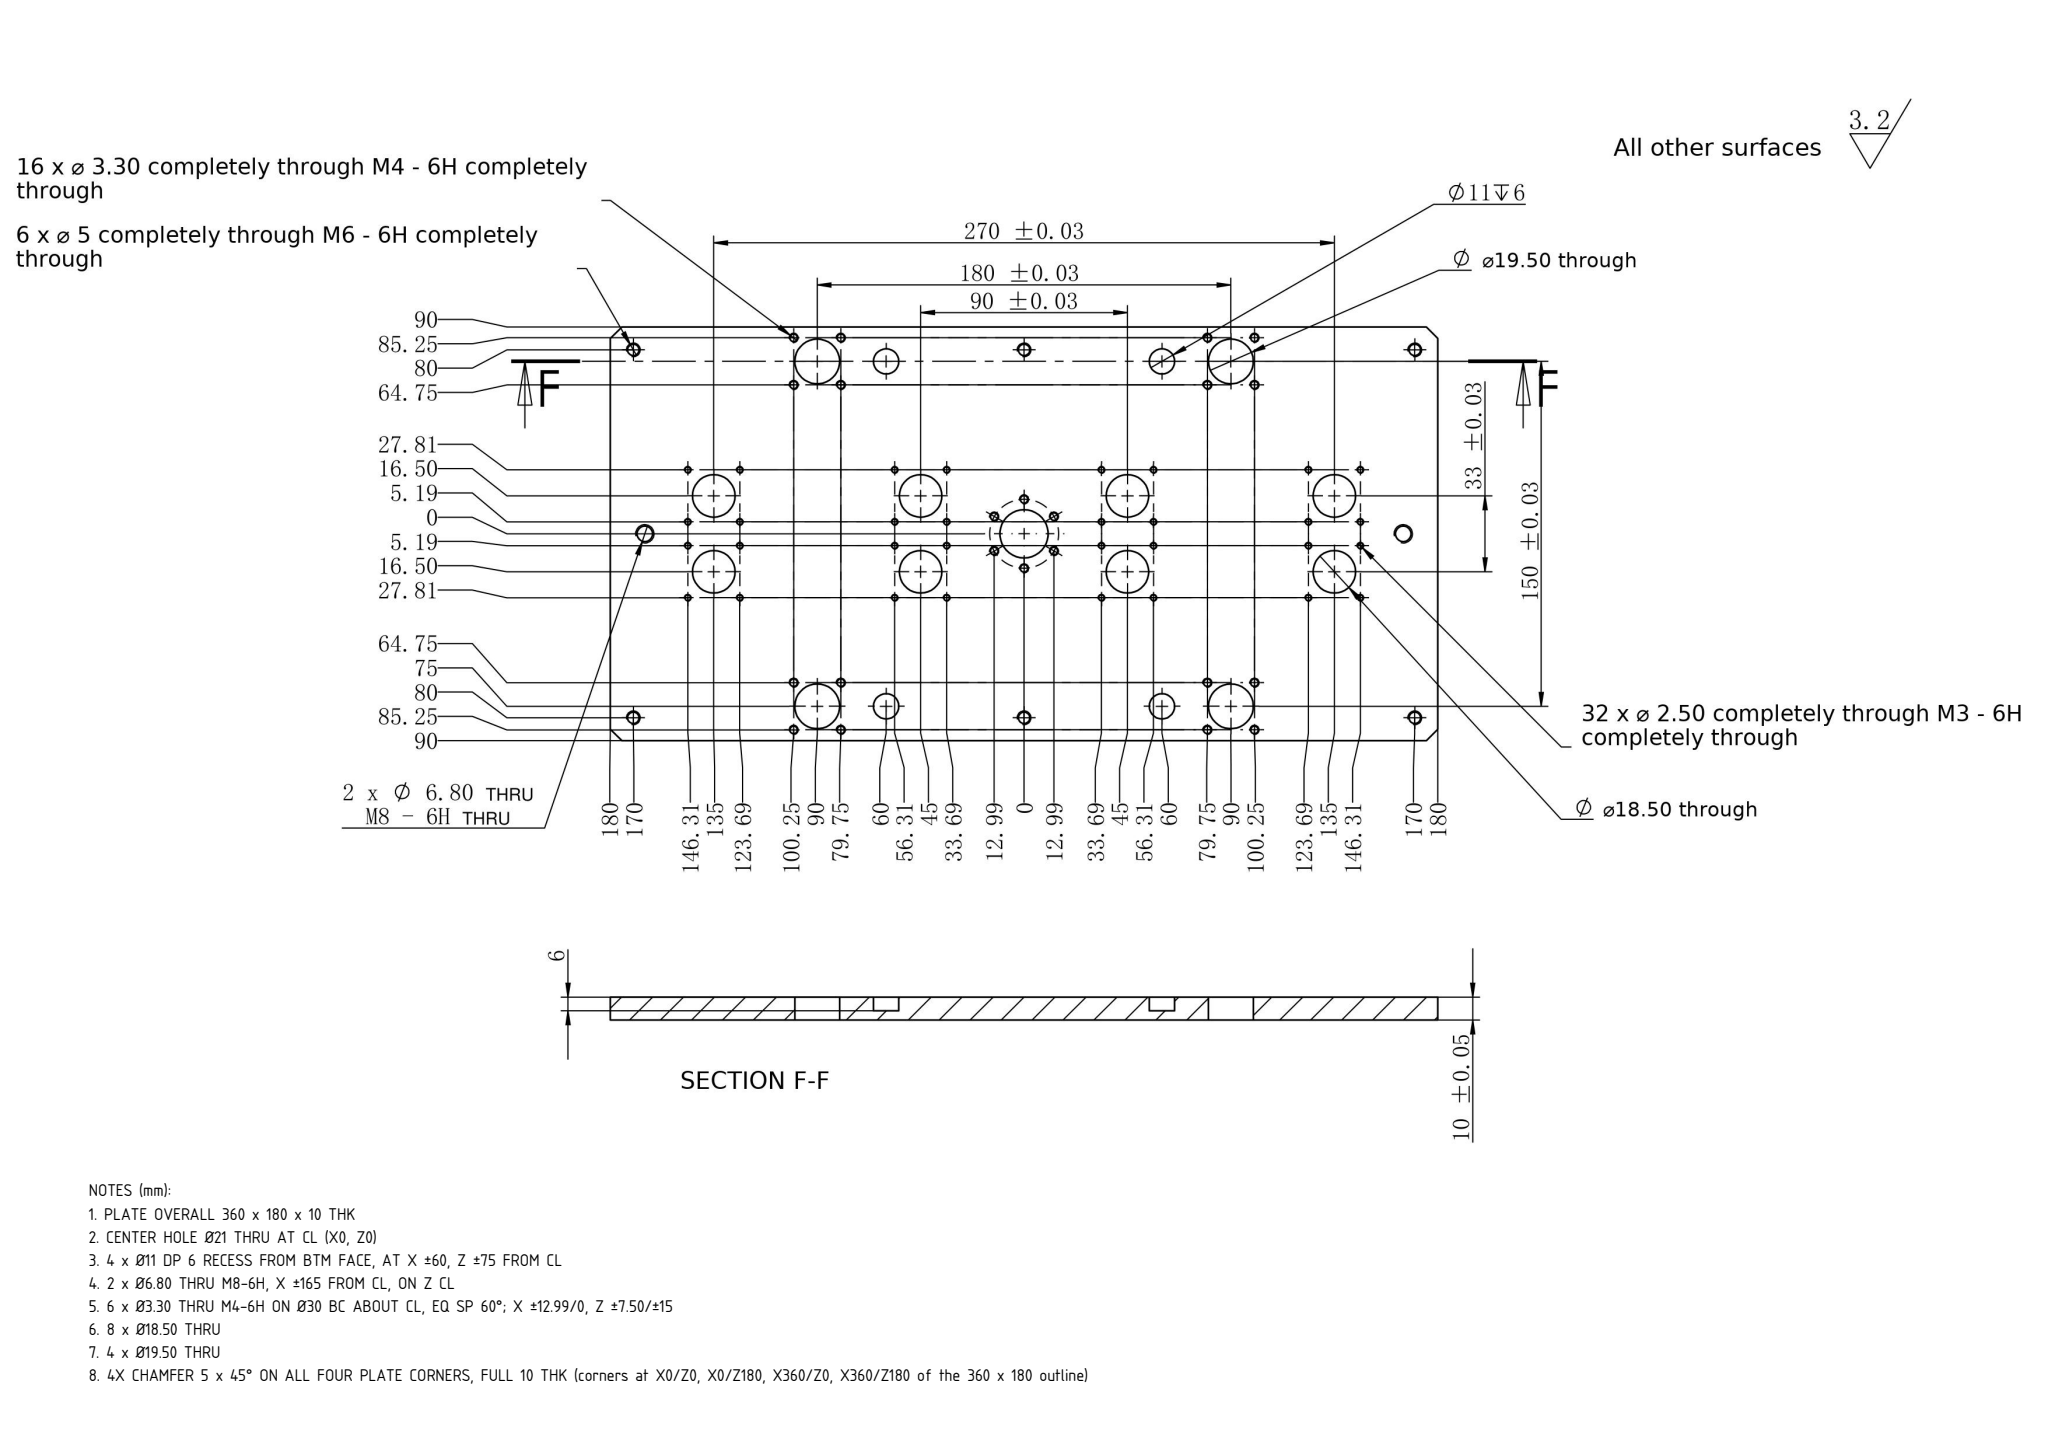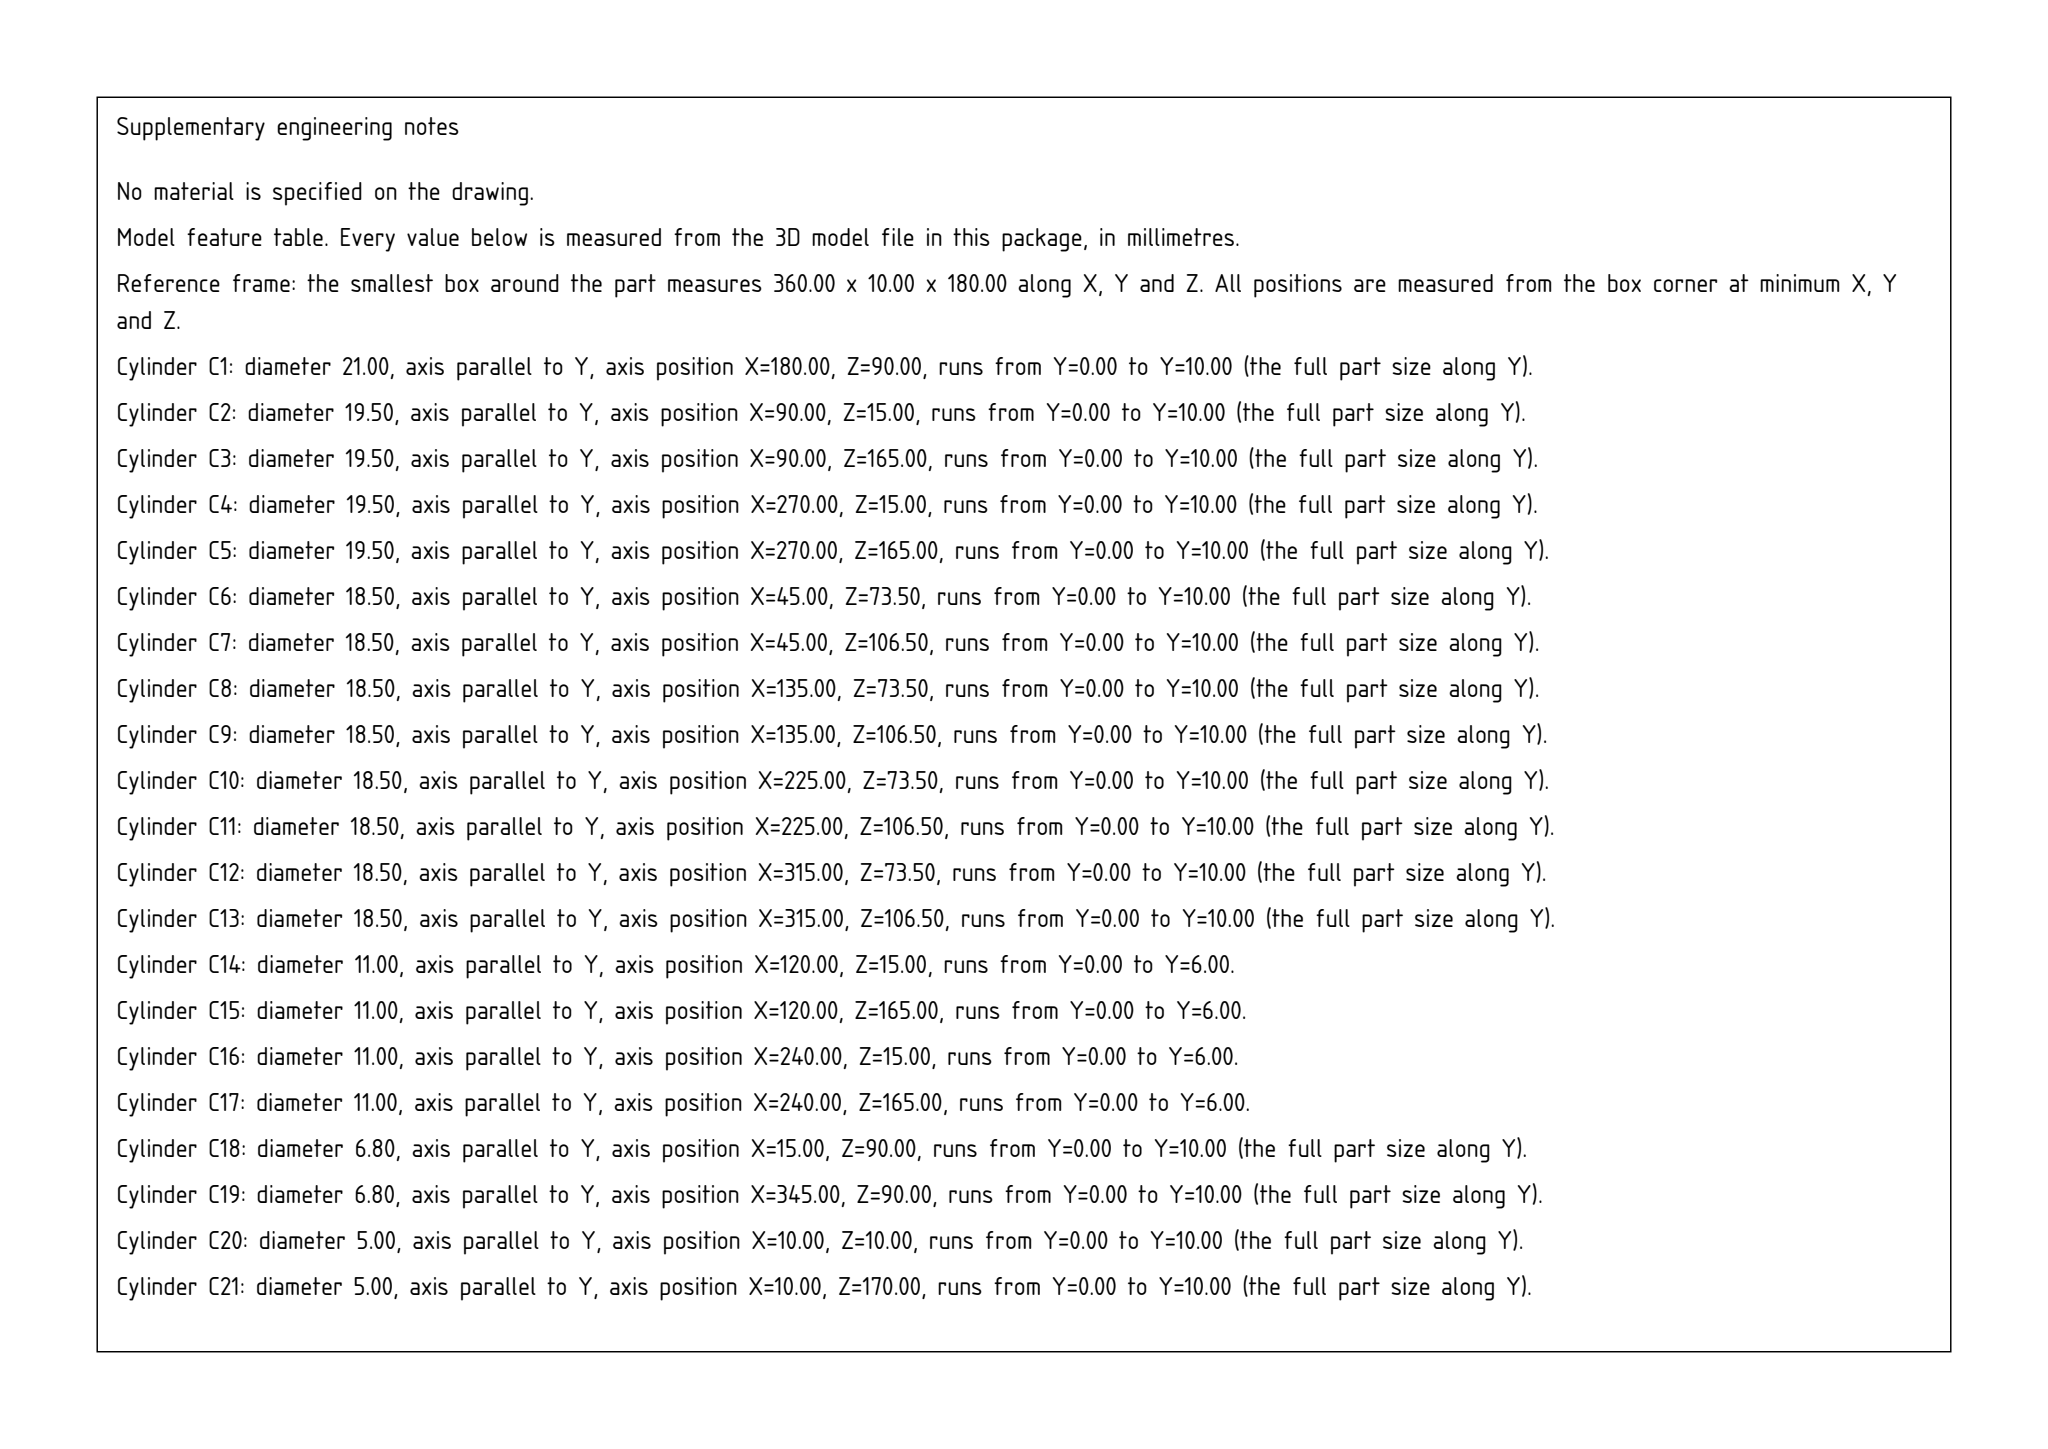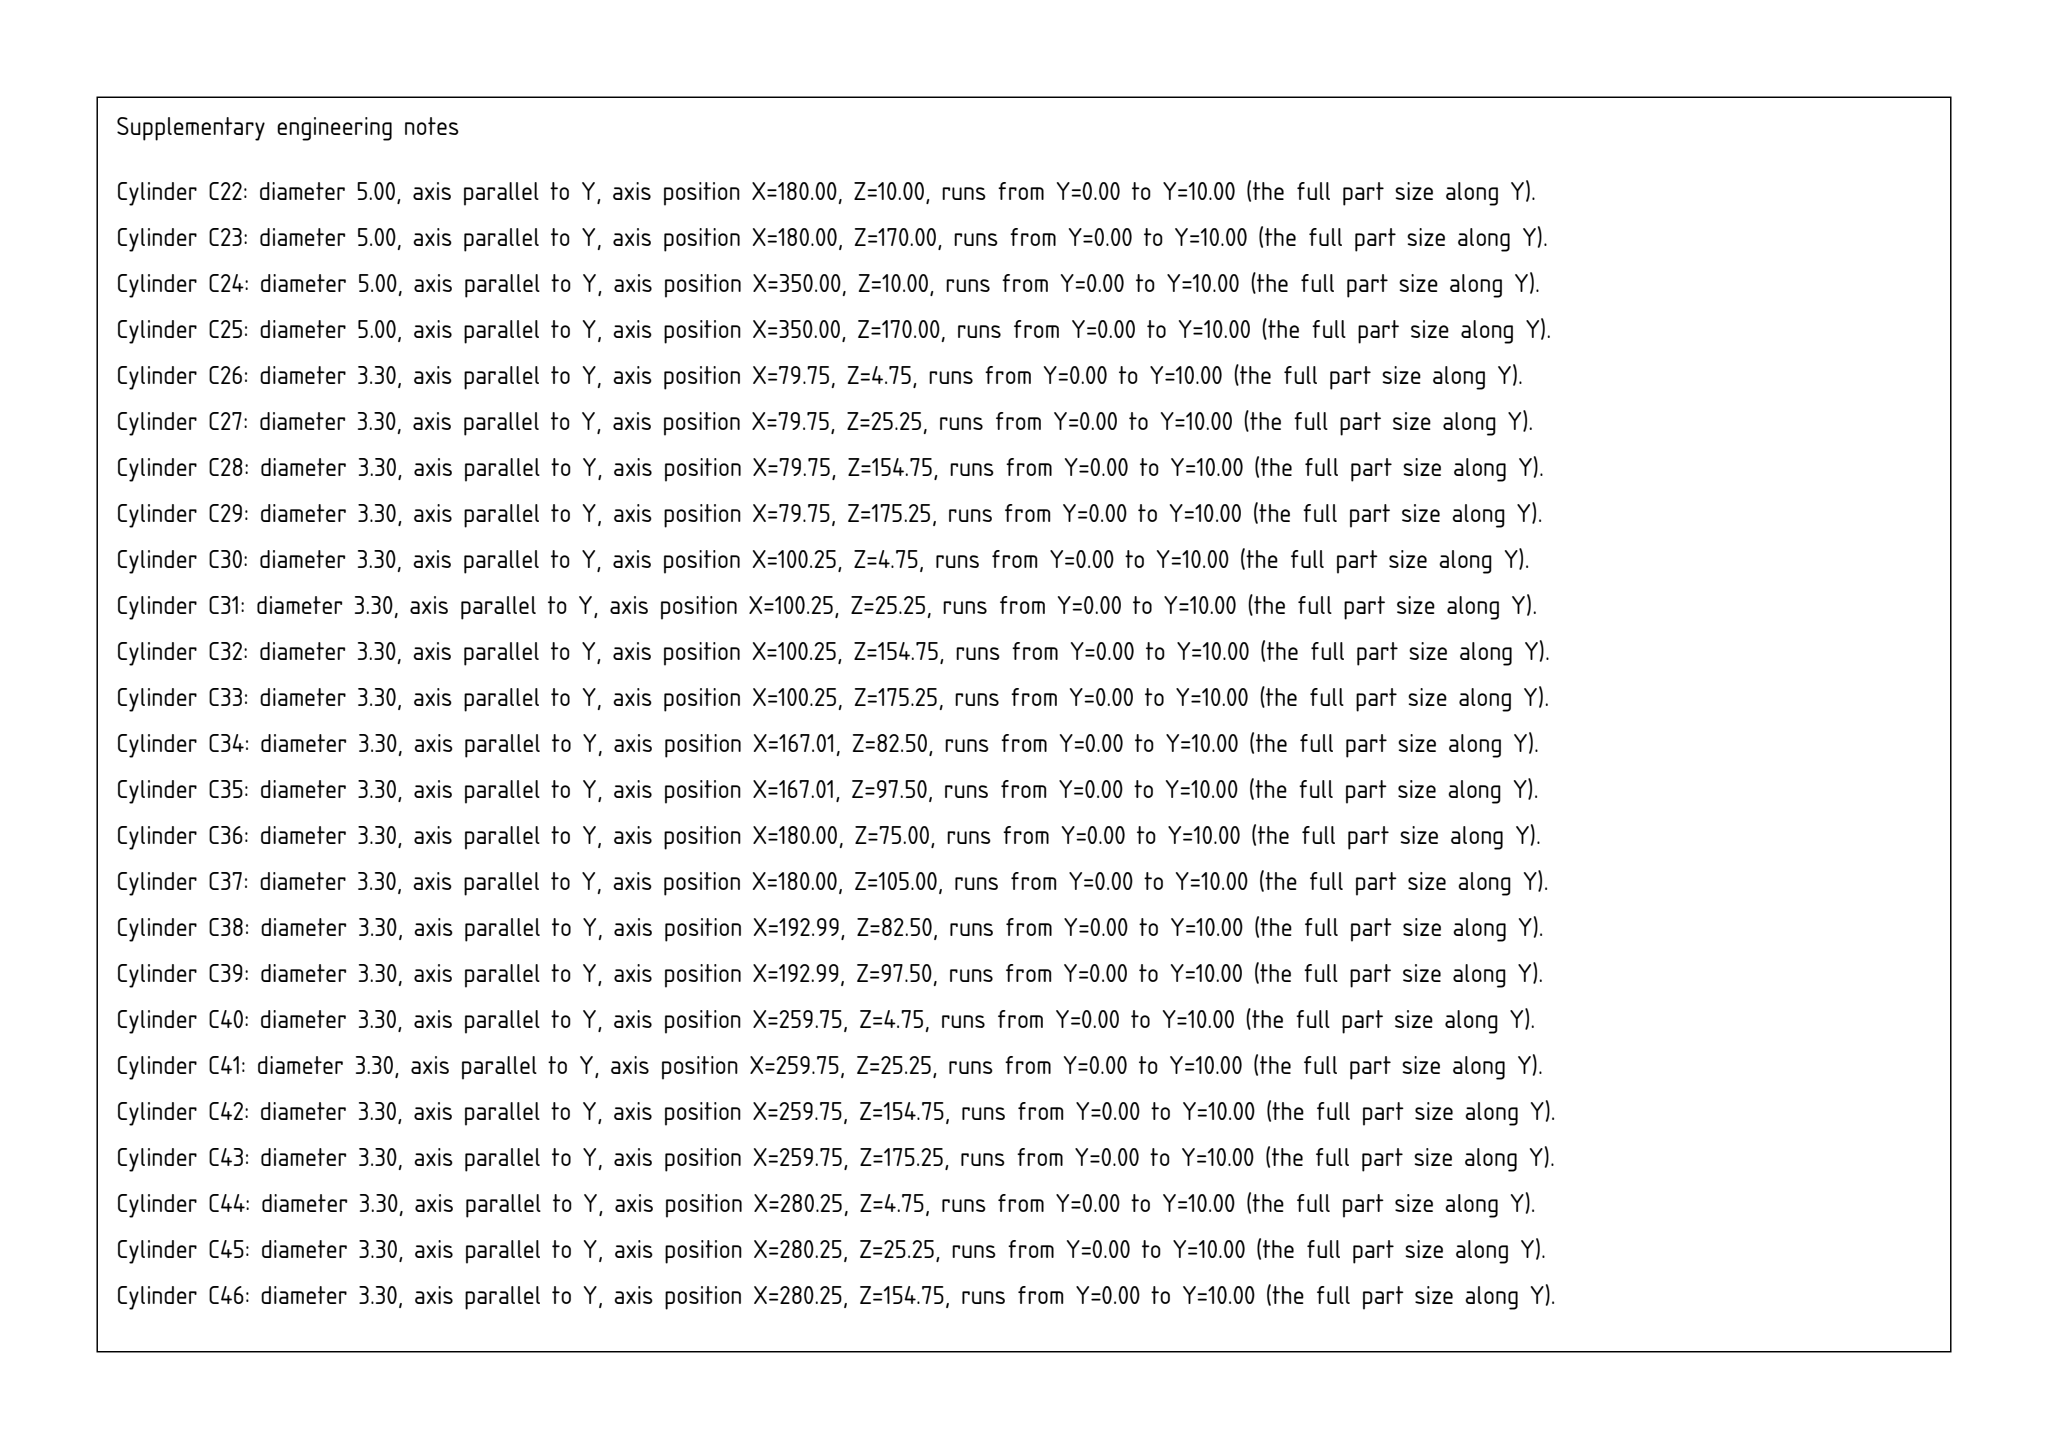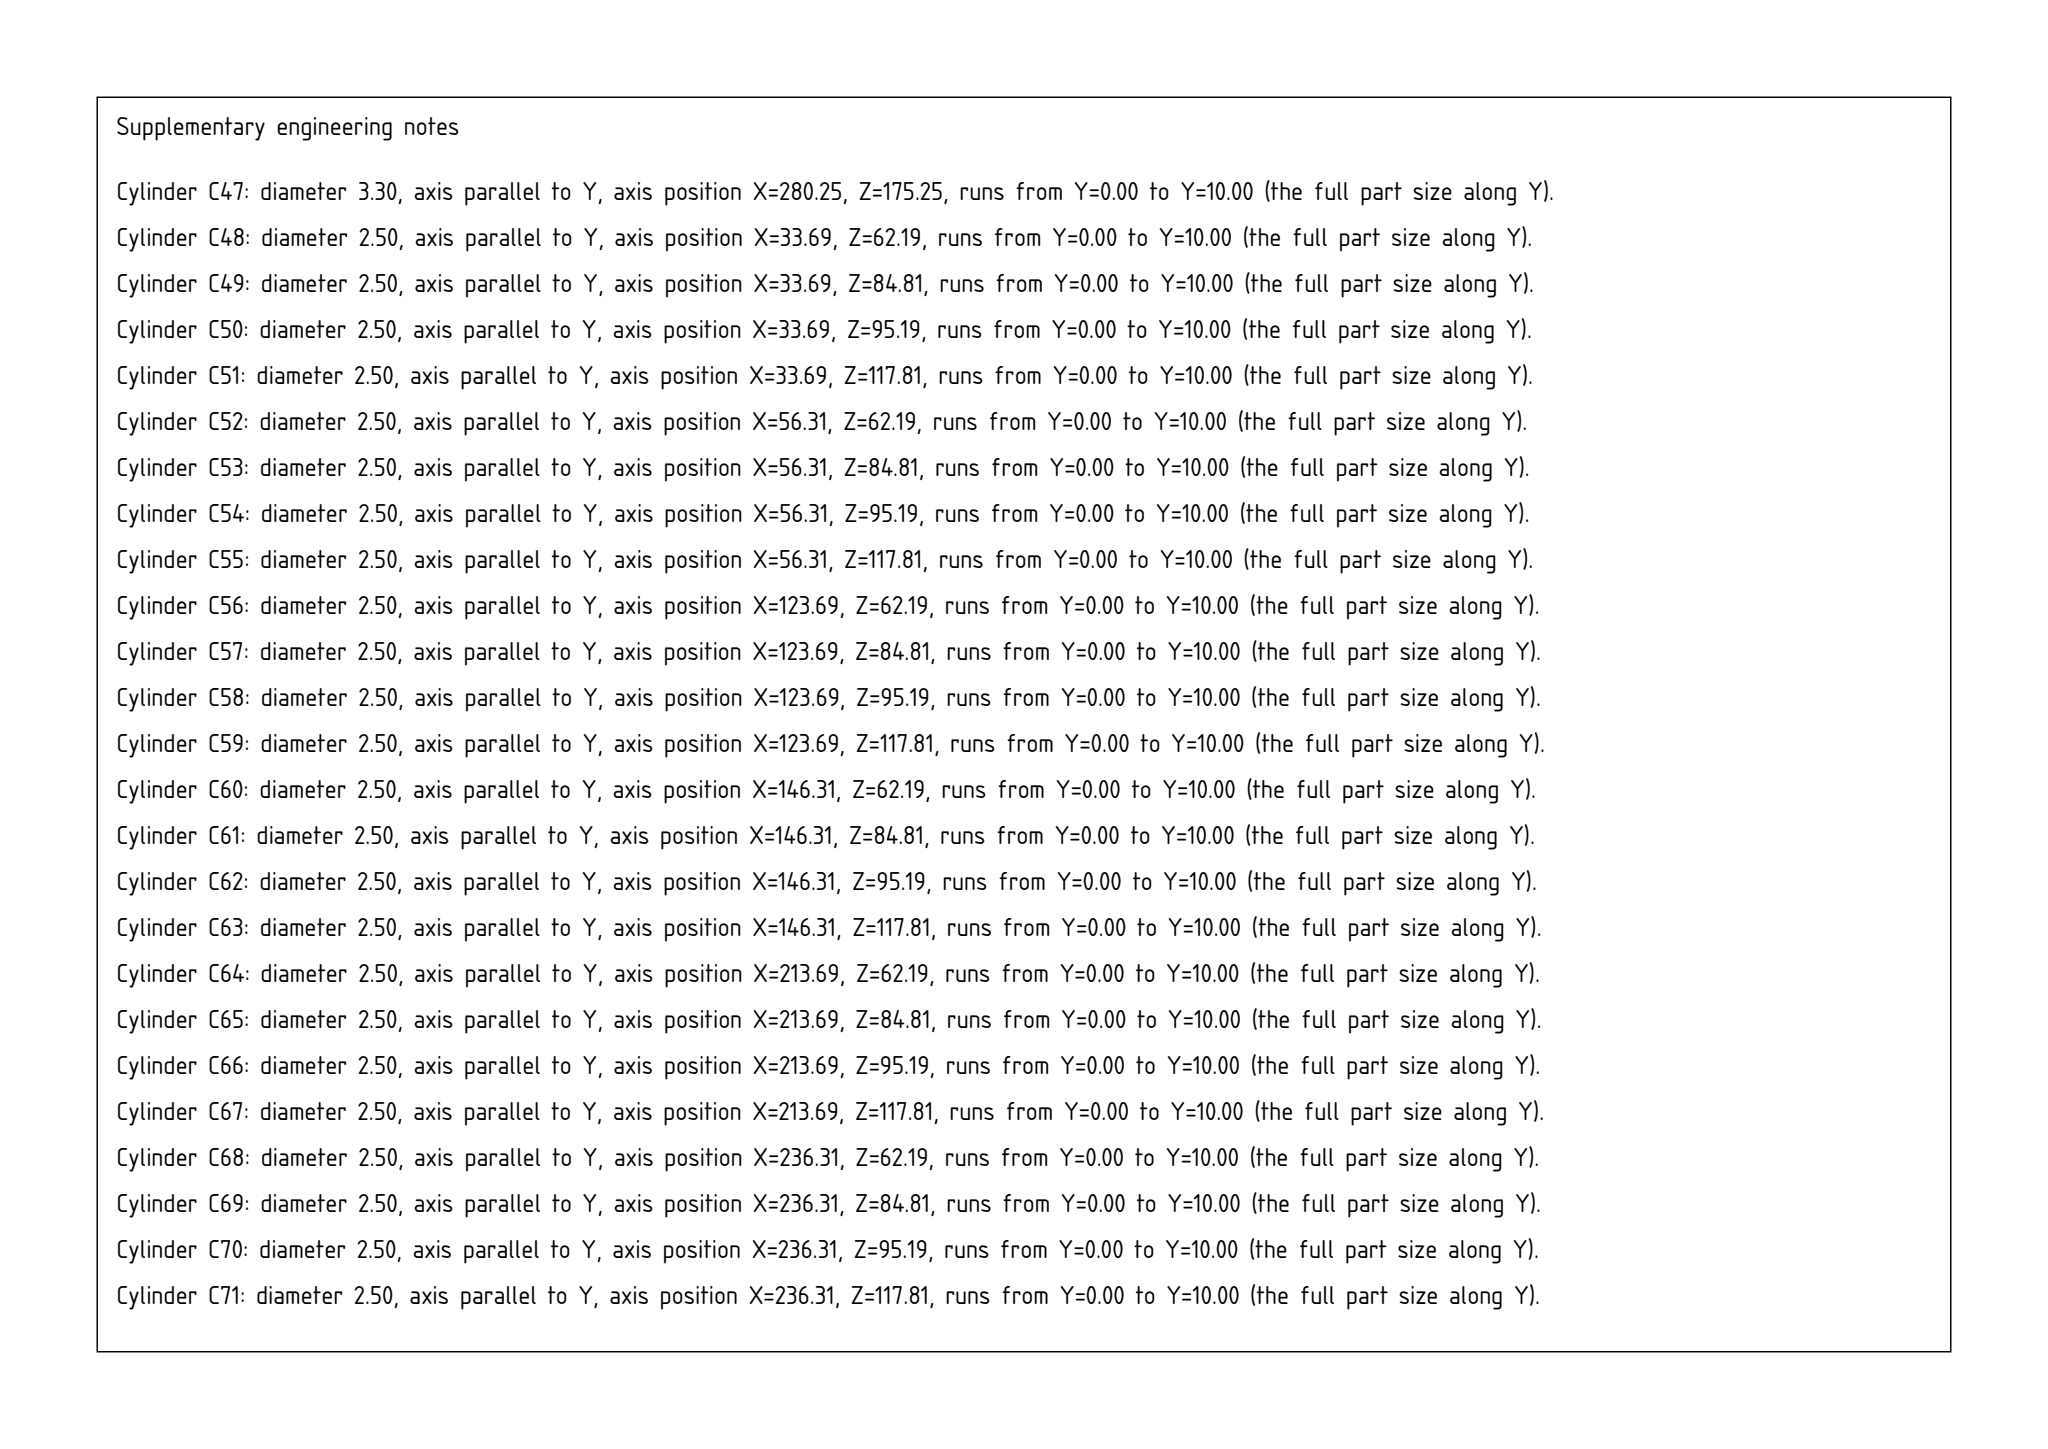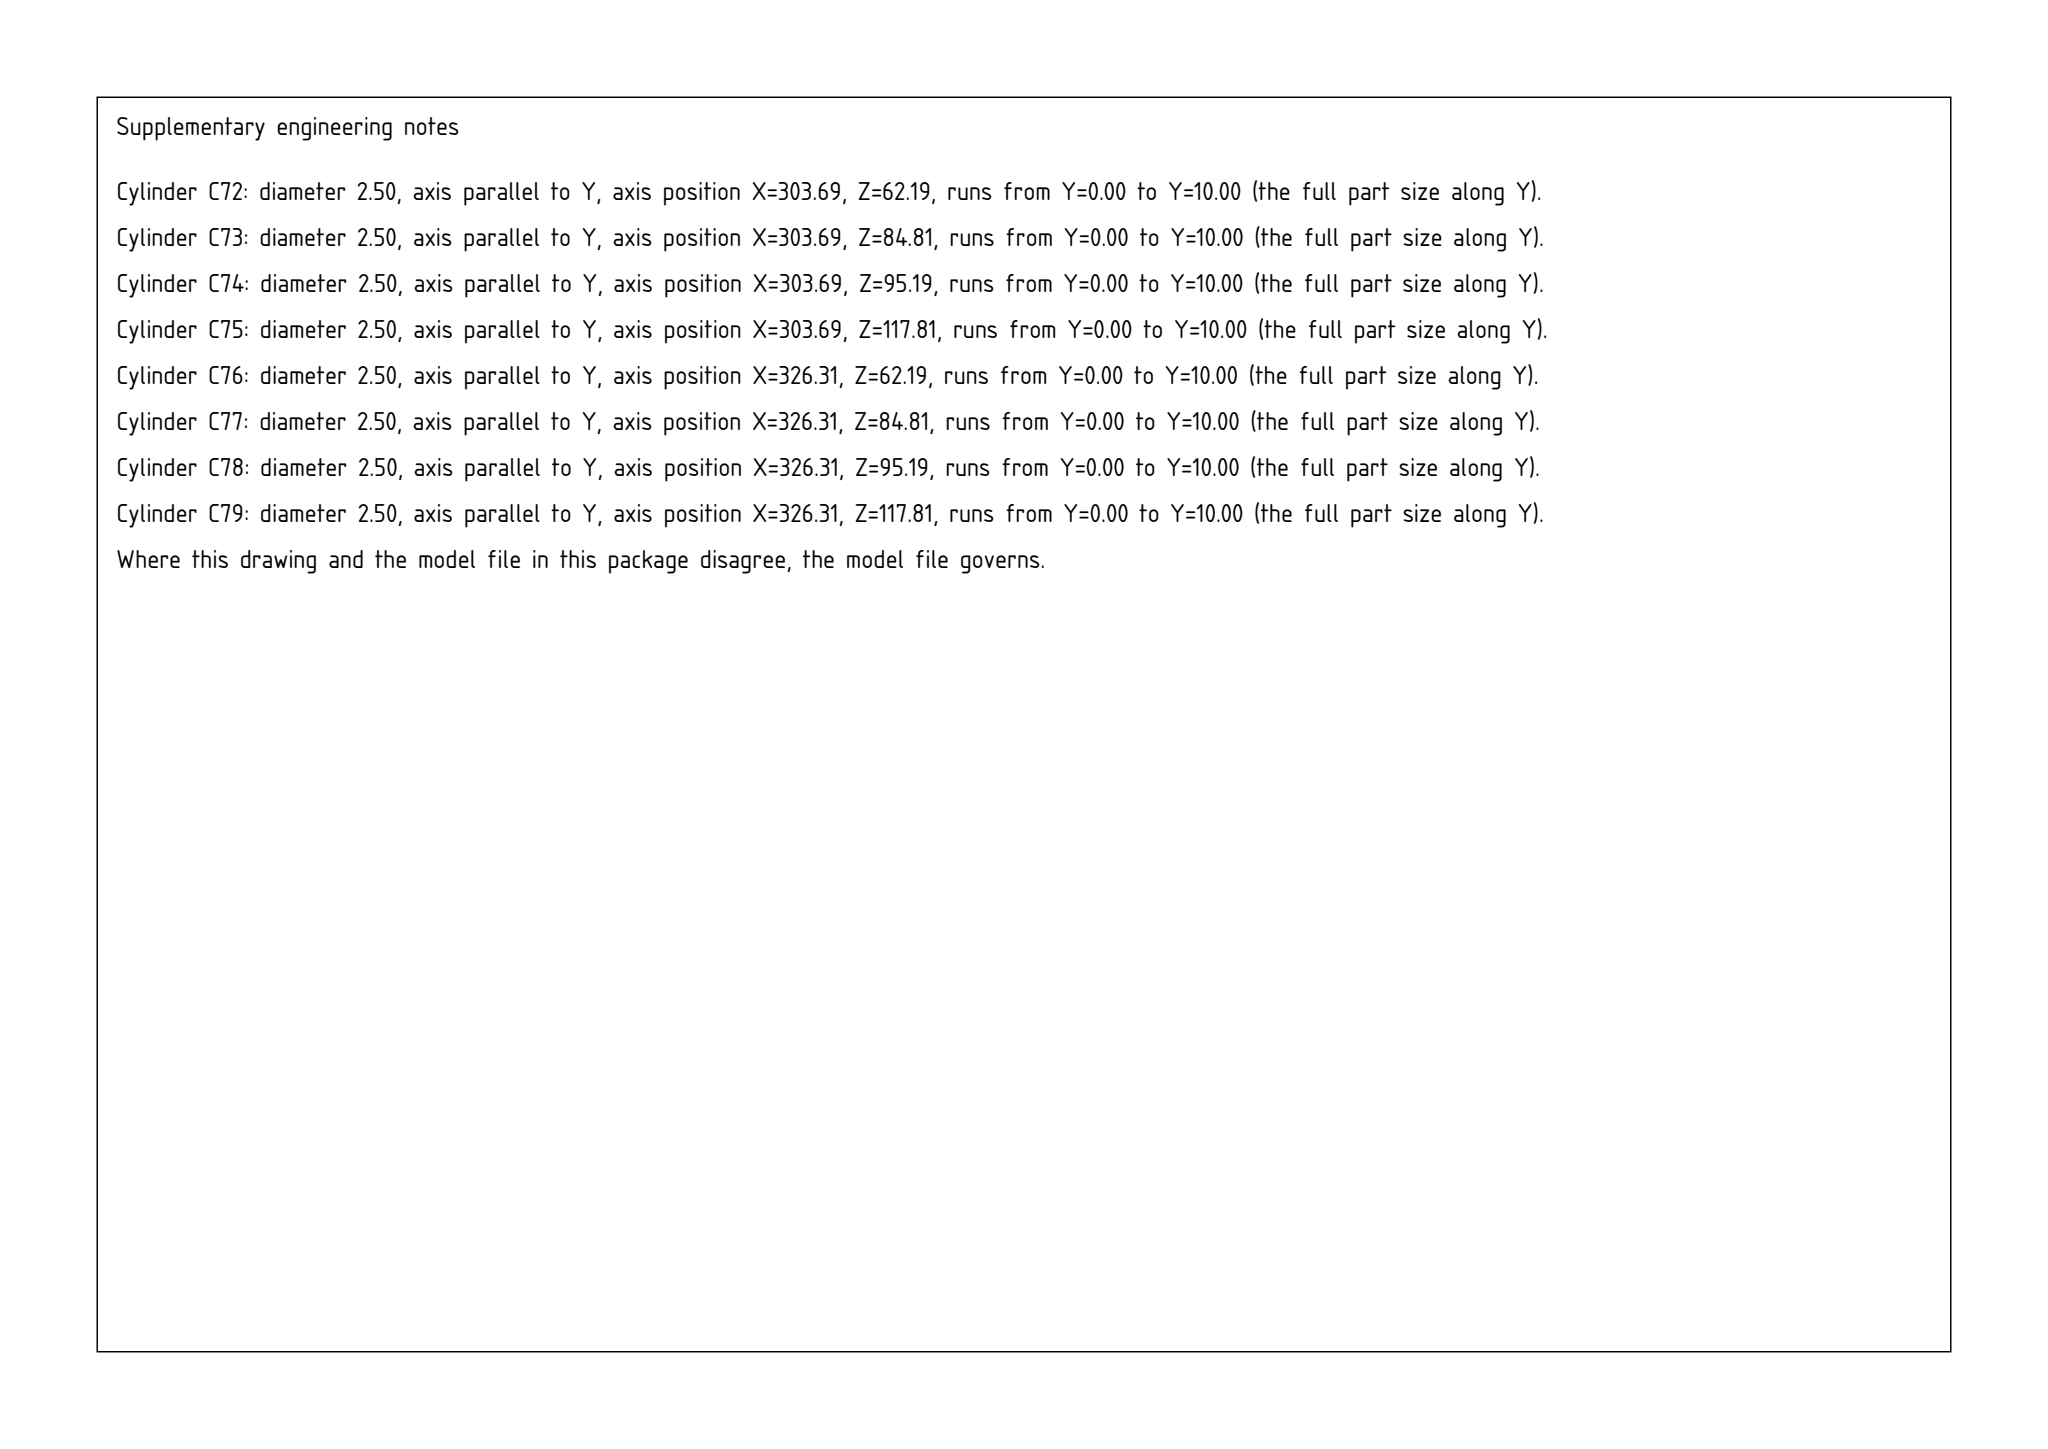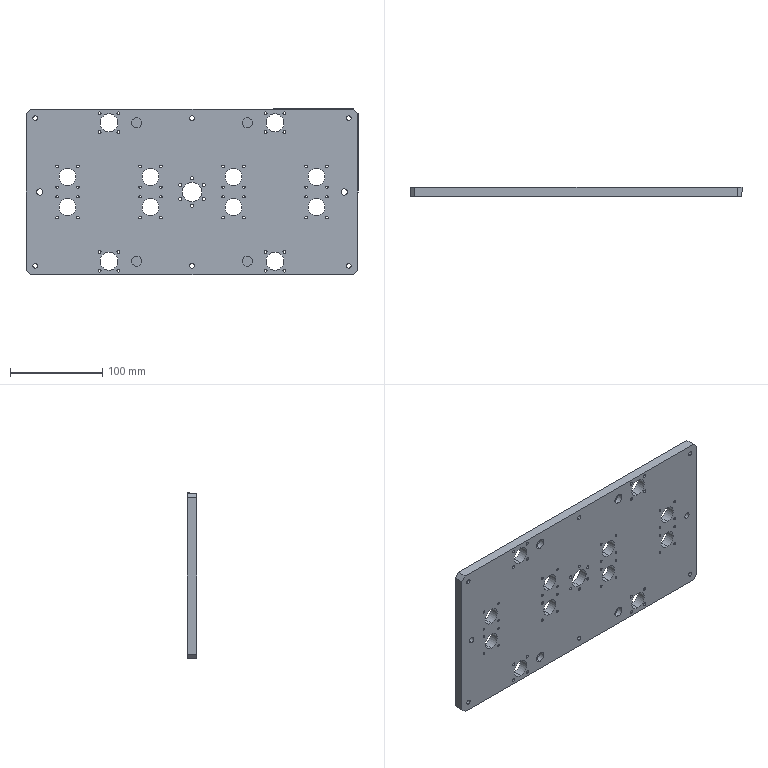Part | SolidWorks | mm | 1 solid | 172 faces | box 360 x 10 x 180 mm | volume 602949 mm3 | cylinder 158 | plane 14 | commonest cylinder face diameters 2.5 x64 3.3 x44 18.5 x16 5 x12 11 x8 19.5 x8 6.8 x4 21 x2
Drawing notes:
PLATE OVERALL 360 x 180 x 10 THK | from the solid: bbox_xyz [360,10,180]; z-planes 0/180, x-planes 0/360, y-planes 0/10
CENTER HOLE Ø21 THRU AT CL (X0, Z0) | from the solid: cyl dia 21, axis y, pos (180,90) = bbox center, len 10 = full thk
4 x Ø11 DP 6 RECESS FROM BTM FACE, AT X ±60, Z ±75 FROM CL | from the solid: cyl dia 11 axis y at (120,15)(120,165)(240,15)(240,165), len 6; y-plane 6.0 count 4
2 x Ø6.80 THRU M8-6H, X ±165 FROM CL, ON Z CL | from the solid: Ø6.8 holes at x=15 & 345 (±165 from CL x=180), z=90 = CL, len 10
6 x Ø3.30 THRU M4-6H ON Ø30 BC ABOUT CL, EQ SP 60°; X ±12.99/0, Z ±7.50/±15 | from the solid: Ø3.3 at (167.01,82.5)(167.01,97.5)(180,75)(180,105)(192.99,82.5)(192.99,97.5), R15 from (180,90)
8 x Ø18.50 THRU | from the solid: 8 cylinders dia 18.5, axis y, len 10 at x=45,135,225,315 / z=73.5,106.5
4 x Ø19.50 THRU | from the solid: 4 cylinders dia 19.5, axis y, len 10 at (90,15),(90,165),(270,15),(270,165)
4X CHAMFER 5 x 45° ON ALL FOUR PLATE CORNERS, FULL 10 THK (corners at X0/Z0, X0/Z180, X360/Z0, X360/Z180 of the 360 x 180 outline) | from the solid: inclined_planes(chamfers/angled faces): 4 faces at angle_to_xyz_axes [45,90,45], size [5,10,5], bbox_from [0,0,0], [0,0,175], [355,0,0], [355,0,175]; axis_planes x=0 and x=360 extent z 5..175, z=0 and z=180 extent x 5..355
build123d program:
from build123d import *

# Parameters (mm, degrees)
SKETCH1_W                  = 360
SKETCH1_H                  = 180
BOSS_EXTRUDE1_DEPTH        = 10
SKETCH2_R                  = 9.25
CUT_EXTRUDE1_DEPTH         = 202.494
CHAMFER1_SIZE              = 5
M6_TAPPED_HOLE1_D          = 5
SKETCH5_R                  = 9.75
CUT_EXTRUDE2_DEPTH         = 202.494
F_21_0_21_DIAMETER_HOLE1_D = 21
M4_TAPPED_HOLE1_D          = 3.3
CIRPATTERN1_COUNT          = 6
SKETCH10_R                 = 5.5
CUT_EXTRUDE3_DEPTH         = 6
M4_TAPPED_HOLE2_D          = 3.3
LPATTERN1_COUNT            = 2
LPATTERN1_PITCH            = 180
LPATTERN1_COUNT_DIR2       = 2
LPATTERN1_PITCH_DIR2       = 150
M3_TAPPED_HOLE1_D          = 2.5
LPATTERN2_COUNT            = 4
LPATTERN2_PITCH            = 90
LPATTERN2_COUNT_DIR2       = 2
LPATTERN2_PITCH_DIR2       = 33
M8_TAPPED_HOLE1_D          = 6.8


with BuildPart() as part:
    # Sketch1 → Boss-Extrude1 (new body)
    with BuildSketch(Plane(origin=(0, 0, 0), x_dir=(1, 0, 0), z_dir=(0, 1, 0))):
        Rectangle(SKETCH1_W, SKETCH1_H)
    extrude(amount=BOSS_EXTRUDE1_DEPTH)

    # Sketch2 → Cut-Extrude1 (cut, through all)
    with BuildSketch(Plane(origin=(0, 10, 0), x_dir=(1, 0, 0), z_dir=(0, 1, 0))):
        with Locations(Location((-135, 16.5, 0), (0, 0, 270))):
            Circle(SKETCH2_R)
        with Locations(Location((-135, -16.5, 0), (0, 0, 270))):
            Circle(SKETCH2_R)
        with Locations(Location((-45, 16.5, 0), (0, 0, 270))):
            Circle(SKETCH2_R)
        with Locations(Location((-45, -16.5, 0), (0, 0, 270))):
            Circle(SKETCH2_R)
        with Locations(Location((45, 16.5, 0), (0, 0, 270))):
            Circle(SKETCH2_R)
        with Locations(Location((45, -16.5, 0), (0, 0, 270))):
            Circle(SKETCH2_R)
        with Locations(Location((135, -16.5, 0), (0, 0, 270))):
            Circle(SKETCH2_R)
        with Locations(Location((135, 16.5, 0), (0, 0, 270))):
            Circle(SKETCH2_R)
    extrude(amount=-CUT_EXTRUDE1_DEPTH, mode=Mode.SUBTRACT)

    # Chamfer1
    chamfer1_edges = [part.edges().sort_by_distance(p)[0] for p in [
        (180, 5, 90),
        (-180, 5, 90),
        (-180, 5, -90),
        (180, 5, -90),
    ]]
    chamfer(chamfer1_edges, length=CHAMFER1_SIZE)

    # M6 Tapped Hole1 (through all)
    with Locations(Plane(origin=(0, 10, 0), x_dir=(1, 0, 0), z_dir=(0, 1, 0))):
        with Locations((170, 80), (0, 80), (-170, 80), (-170, -80), (0, -80), (170, -80)):
            Hole(M6_TAPPED_HOLE1_D / 2)

    # Sketch5 → Cut-Extrude2 (cut, through all)
    with BuildSketch(Plane(origin=(0, 10, 0), x_dir=(1, 0, 0), z_dir=(0, 1, 0))):
        with Locations(Location((90, 75, 0), (0, 0, 270))):
            Circle(SKETCH5_R)
        with Locations(Location((90, -75, 0), (0, 0, 270))):
            Circle(SKETCH5_R)
        with Locations(Location((-90, -75, 0), (0, 0, 270))):
            Circle(SKETCH5_R)
        with Locations(Location((-90, 75, 0), (0, 0, 270))):
            Circle(SKETCH5_R)
    extrude(amount=-CUT_EXTRUDE2_DEPTH, mode=Mode.SUBTRACT)

    # 21.0 _21_ Diameter Hole1 (through all)
    with Locations(Plane(origin=(0, 10, 0), x_dir=(1, 0, 0), z_dir=(0, 1, 0))):
        with Locations((0, 0)):
            Hole(F_21_0_21_DIAMETER_HOLE1_D / 2)

    # M4 Tapped Hole1 (through all)
    with Locations(Plane(origin=(0, 10, 0), x_dir=(1, 0, 0), z_dir=(0, 1, 0))):
        with Locations((0, 15)):
            m4_tapped_hole1 = Hole(M4_TAPPED_HOLE1_D / 2)

    # CirPattern1: M4 Tapped Hole1 ×6 about axis
    cirpattern1_axis = Axis((0, 0, 0), (0, 1, 0))
    for i in range(1, CIRPATTERN1_COUNT):
        add(m4_tapped_hole1.rotate(cirpattern1_axis, i * 360 / CIRPATTERN1_COUNT), mode=Mode.SUBTRACT)

    # Sketch10 → Cut-Extrude3 (cut)
    with BuildSketch(Plane.XZ):
        with Locations(Location((-60, -75, 0), (0, 0, 270))):
            Circle(SKETCH10_R)
        with Locations(Location((-60, 75, 0), (0, 0, 270))):
            Circle(SKETCH10_R)
        with Locations(Location((60, 75, 0), (0, 0, 270))):
            Circle(SKETCH10_R)
        with Locations(Location((60, -75, 0), (0, 0, 270))):
            Circle(SKETCH10_R)
    extrude(amount=-CUT_EXTRUDE3_DEPTH, mode=Mode.SUBTRACT)

    # M4 Tapped Hole2 (through all)
    with Locations(Plane(origin=(0, 0, 0), x_dir=(-1, 0, 0), z_dir=(0, -1, 0))):
        with Locations((-100.253, 85.253), (-79.747, 85.253), (-79.747, 64.747), (-100.253, 64.747)):
            m4_tapped_hole2 = Hole(M4_TAPPED_HOLE2_D / 2)

    # LPattern1: M4 Tapped Hole2 2 × 2
    with Locations(*[(-i * LPATTERN1_PITCH, 0, j * LPATTERN1_PITCH_DIR2) for i in range(LPATTERN1_COUNT) for j in range(LPATTERN1_COUNT_DIR2) if (i, j) != (0, 0)]):
        add(m4_tapped_hole2, mode=Mode.SUBTRACT)

    # M3 Tapped Hole1 (through all)
    with Locations(Plane(origin=(0, 10, 0), x_dir=(1, 0, 0), z_dir=(0, 1, 0))):
        with Locations((123.686, -5.186), (146.314, -5.186), (146.314, -27.814), (123.686, -27.814)):
            m3_tapped_hole1 = Hole(M3_TAPPED_HOLE1_D / 2)

    # LPattern2: M3 Tapped Hole1 4 × 2
    with Locations(*[(-i * LPATTERN2_PITCH, 0, -j * LPATTERN2_PITCH_DIR2) for i in range(LPATTERN2_COUNT) for j in range(LPATTERN2_COUNT_DIR2) if (i, j) != (0, 0)]):
        add(m3_tapped_hole1, mode=Mode.SUBTRACT)

    # M8 Tapped Hole1 (through all)
    with Locations(Plane(origin=(0, 0, 0), x_dir=(-1, 0, 0), z_dir=(0, -1, 0))):
        with Locations((-165, 0), (165, 0)):
            Hole(M8_TAPPED_HOLE1_D / 2)


solid = part.part